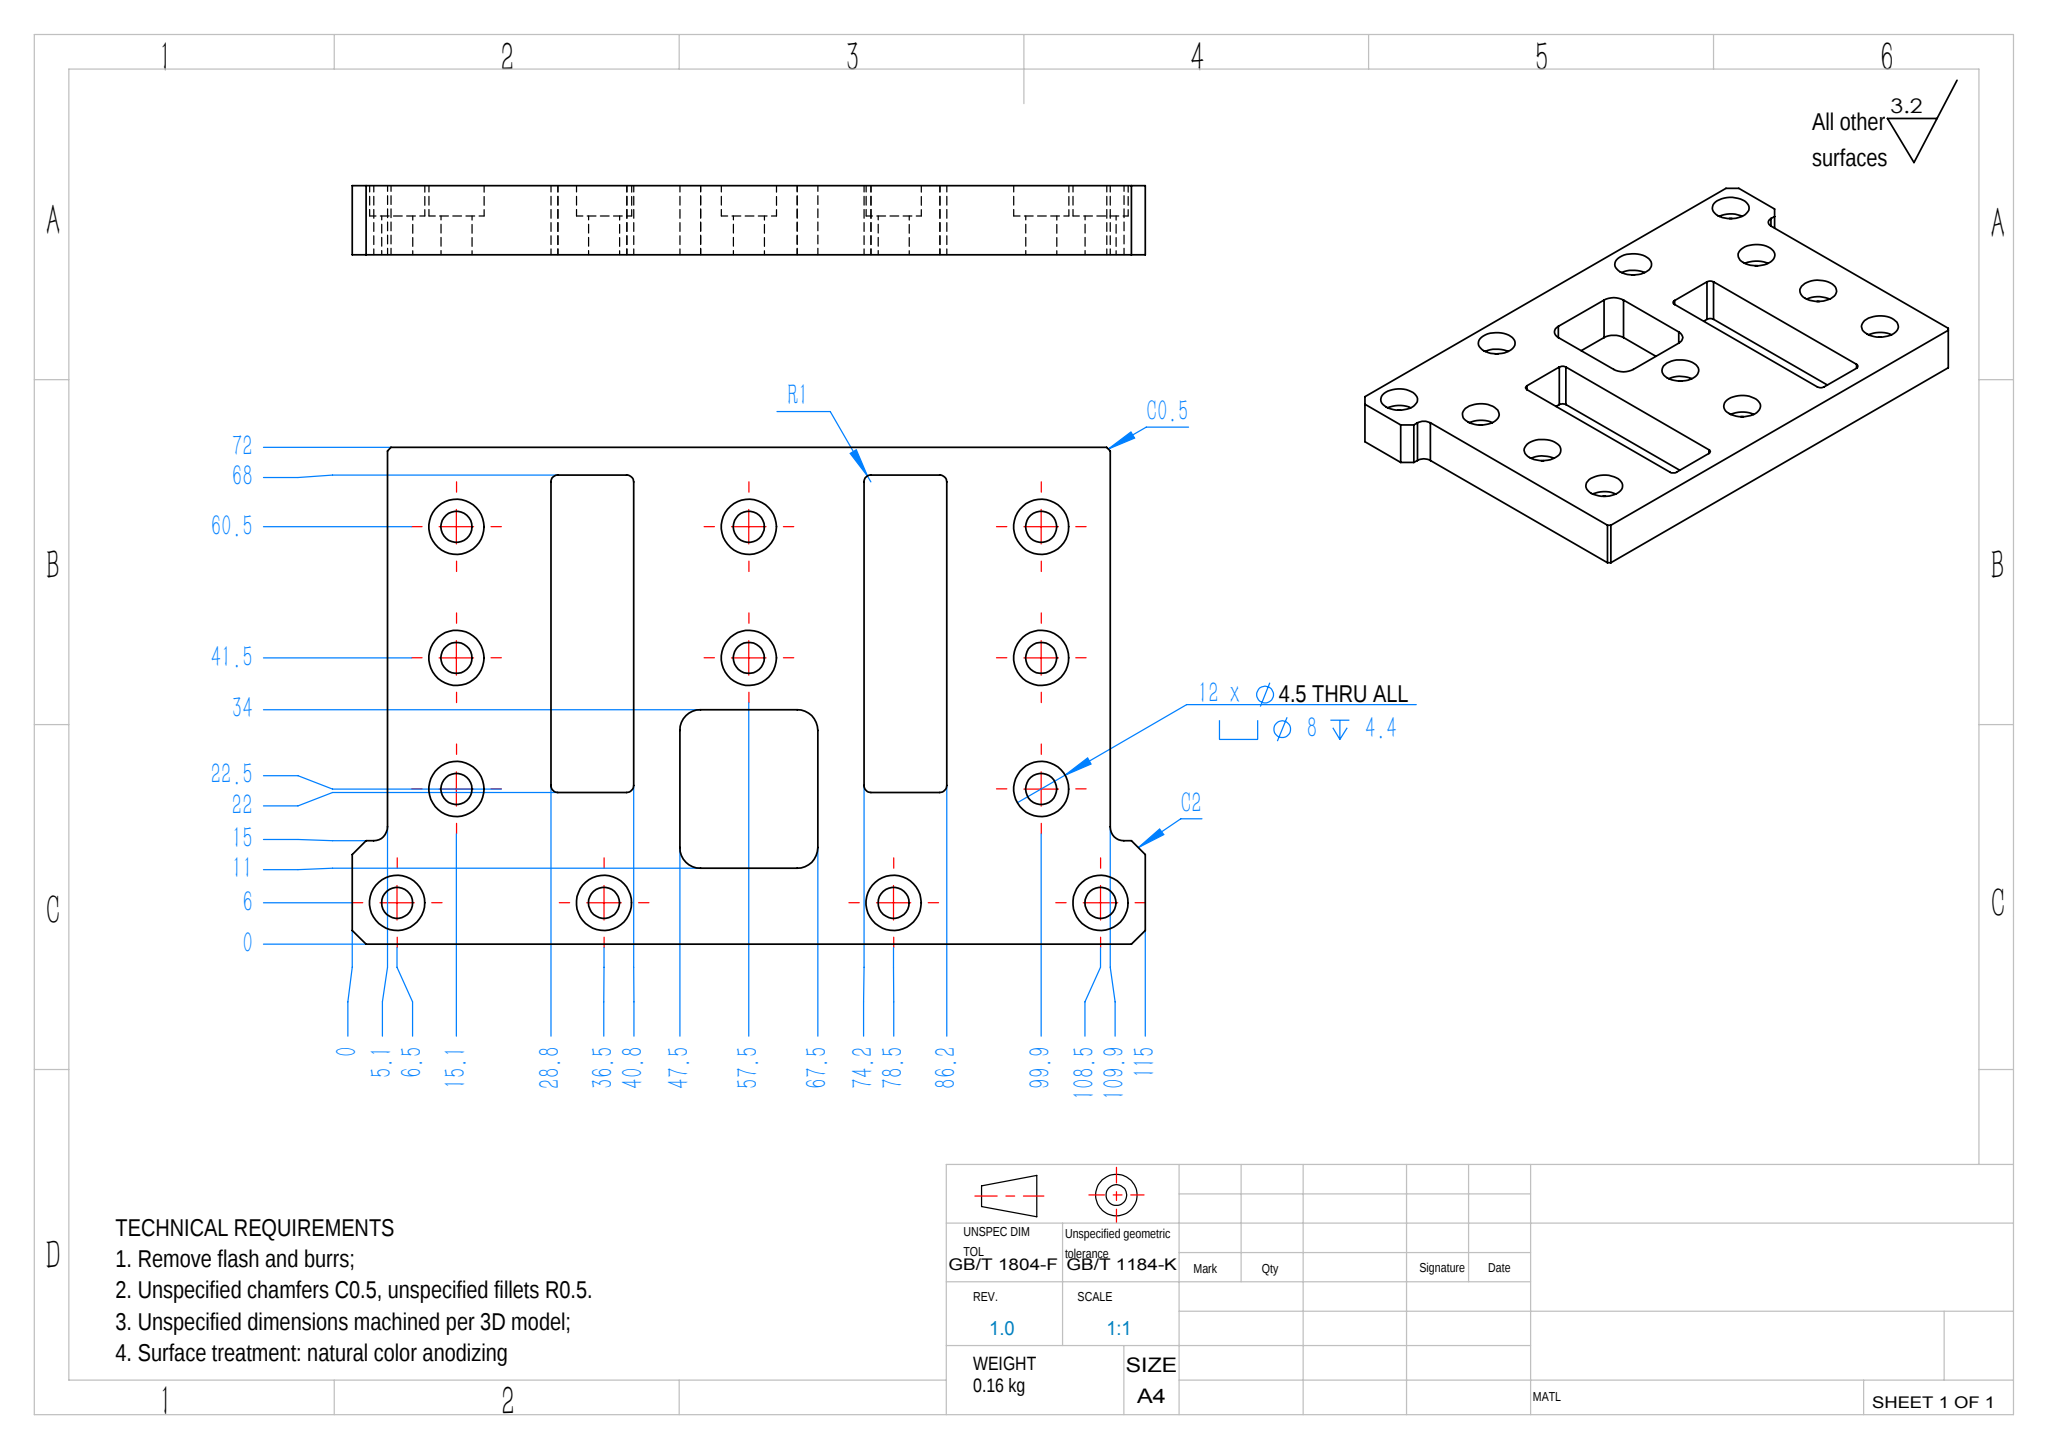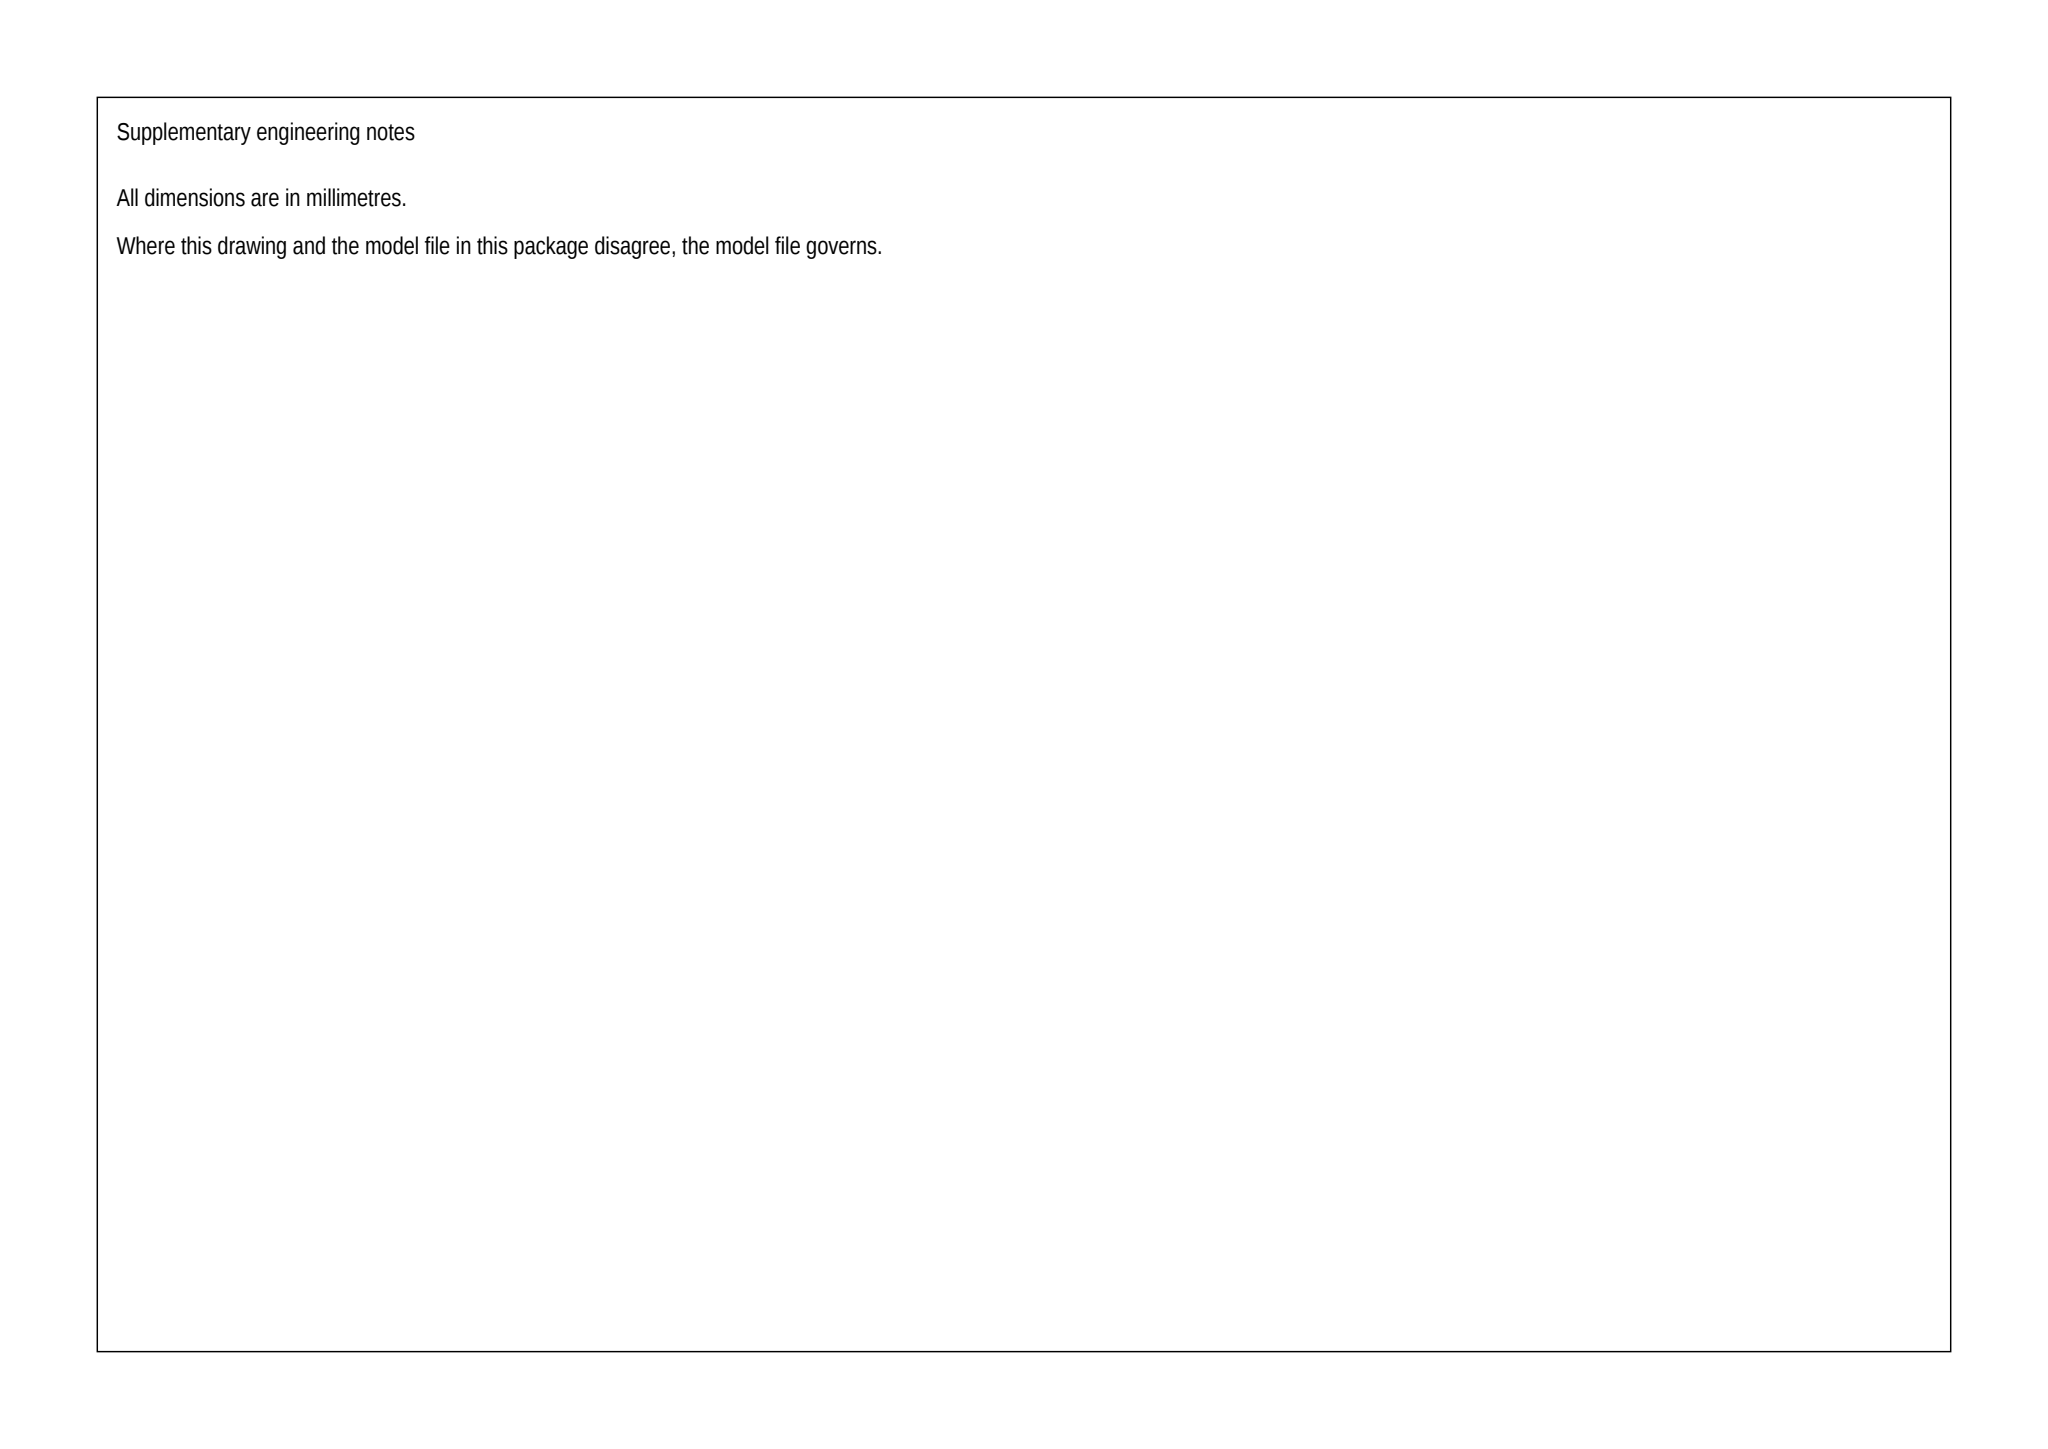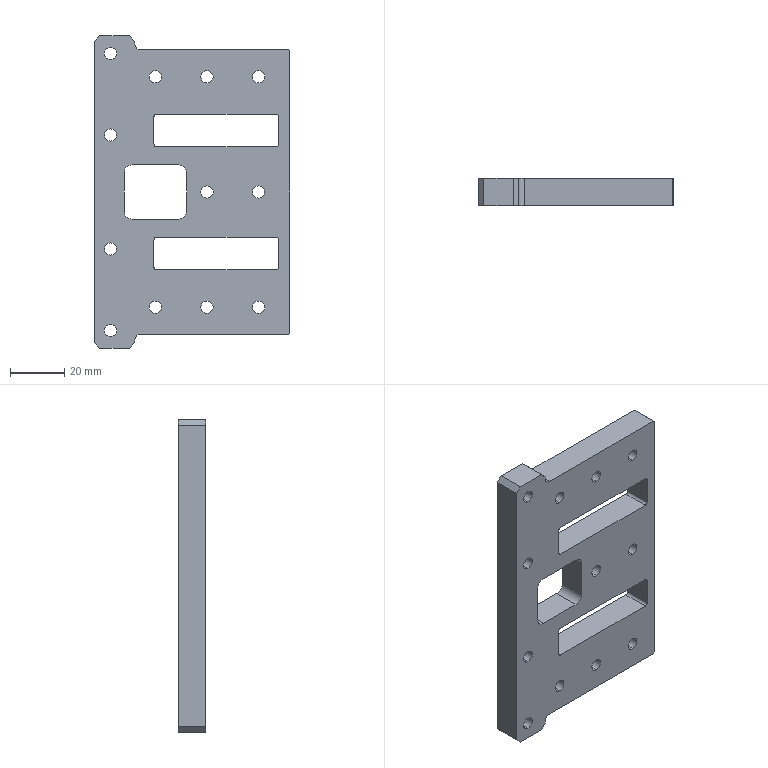Part | SolidWorks | mm | 1 solid | 102 faces | box 72 x 10 x 115 mm | volume 57652 mm3 | cylinder 62 | plane 40 | commonest cylinder face diameters 8 x24 4.5 x24 2 x8 6 x4 4 x2
Drawing notes:
PLATE 115 X 72 X 10 THK | from the solid: bbox_xyz [72,10,115]; y planes only at 0.0 and 10.0
2X EDGE STEP 5.1 DP X 57 HIGH (X15 TO X72), FULL THK | from the solid: z planes 0/5.1 and 109.9/115 (5.1); x planes 15.0 (2) to 72.0 = 57; no mid y plane, full 10 thk
2X R2 AT STEP RE-ENTRANT CNRS (X15 / Z5.1 & Z109.9) | from the solid: Ø4.0 y-axis cyls at (x17,z3.1) and (x17,z111.9), L=10, tangent to x=15 and z=5.1/109.9
C2 AT STEP CNR (X15/Z0 & X15/Z115), 2X | from the solid: C2 called out on sheet 1 at X15/Z115; mirrored x=15 (2) / z=0 & 115 step geometry at both ends
2X SLOT 12 WIDE X 46 LG, R1 ENDS, THRU 10 | from the solid: z planes 28.8/40.8 and 74.2/86.2 = 12 wide; x planes 22/68 = 46 lg; R1 end cyls Ø2 L=10
RND RECT POCKET 23 X 20, R3 CNRS, THRU 10 | from the solid: x planes 11/34 = 23; z planes 47.5/67.5 = 20; Ø6 cnr cyls at x14/31, z50.5/64.5, L=10
build123d program:
from build123d import *

# Parameters (mm, degrees)
SKETCH2_W                                       = 72
SKETCH2_H                                       = 115
BOSS_EXTRUDE1_DEPTH                             = 5
CUT_EXTRUDE3_DEPTH                              = 20
CHAMFER1_SIZE                                   = 2
SKETCH11_W                                      = 57
SKETCH11_H                                      = 5.1
CUT_EXTRUDE4_DEPTH                              = 69.573
M4_HEX_SOCKET_HEAD_CAP_SCREW_CBORE1_D           = 4.5
M4_HEX_SOCKET_HEAD_CAP_SCREW_CBORE1_CBORE_D     = 8
M4_HEX_SOCKET_HEAD_CAP_SCREW_CBORE1_CBORE_DEPTH = 4.4
CHAMFER2_SIZE                                   = 2
CHAMFER3_SIZE                                   = 0.5
FILLET1_R                                       = 2
SKETCH12_W                                      = 23
SKETCH12_H                                      = 20
CUT_EXTRUDE5_DEPTH                              = 69.573
FILLET2_R                                       = 3


with BuildPart() as part:
    # Sketch2 → Boss-Extrude1 (new, symmetric)
    with BuildSketch(Plane(origin=(0, 0, 0), x_dir=(1, 0, 0), z_dir=(0, 1, 0))):
        Rectangle(SKETCH2_W, SKETCH2_H)
    extrude(amount=BOSS_EXTRUDE1_DEPTH, both=True)

    # Sketch5 → Cut-Extrude3 (cut)
    with BuildSketch(Plane.XZ.offset(5)):
        with BuildLine():
            Line((31, -16.7), (-13, -16.7))
            ThreePointArc((-13, -16.7), (-13.707, -16.993), (-14, -17.7))
            Line((-14, -17.7), (-14, -27.7))
            ThreePointArc((-14, -27.7), (-13.707, -28.407), (-13, -28.7))
            Line((-13, -28.7), (31, -28.7))
            ThreePointArc((31, -28.7), (31.707, -28.407), (32, -27.7))
            Line((32, -27.7), (32, -17.7))
            ThreePointArc((32, -17.7), (31.707, -16.993), (31, -16.7))
        make_face()
        with BuildLine():
            Line((-14, 17.7), (-14, 27.7))
            ThreePointArc((-14, 27.7), (-13.707, 28.407), (-13, 28.7))
            Line((-13, 28.7), (31, 28.7))
            ThreePointArc((31, 28.7), (31.707, 28.407), (32, 27.7))
            Line((32, 27.7), (32, 17.7))
            ThreePointArc((32, 17.7), (31.707, 16.993), (31, 16.7))
            Line((31, 16.7), (-13, 16.7))
            ThreePointArc((-13, 16.7), (-13.707, 16.993), (-14, 17.7))
        make_face()
    extrude(amount=-CUT_EXTRUDE3_DEPTH, mode=Mode.SUBTRACT)

    # Chamfer1
    chamfer1_edges = [part.edges().sort_by_distance(p)[0] for p in [
        (-36, 0, 57.5),
        (-36, 0, -57.5),
    ]]
    chamfer(chamfer1_edges, length=CHAMFER1_SIZE)

    # Sketch11 → Cut-Extrude4 (cut, through all)
    with BuildSketch(Plane.XZ.offset(5)):
        with Locations((7.5, 54.95)):
            Rectangle(SKETCH11_W, SKETCH11_H)
        with Locations((7.5, -54.95)):
            Rectangle(SKETCH11_W, SKETCH11_H)
    extrude(amount=-CUT_EXTRUDE4_DEPTH, mode=Mode.SUBTRACT)

    # M4 Hex Socket Head Cap Screw CBORE1 (through all)
    with Locations(Plane(origin=(0, 5, 0), x_dir=(1, 0, 0), z_dir=(0, 1, 0))):
        with Locations((5.5, 42.4), (24.5, 42.4), (-13.5, 42.4), (-30, 51), (5.5, 0), (24.5, 0), (-30, 21), (5.5, -42.4), (24.5, -42.4), (-13.5, -42.4), (-30, -21), (-30, -51)):
            CounterBoreHole(M4_HEX_SOCKET_HEAD_CAP_SCREW_CBORE1_D / 2, M4_HEX_SOCKET_HEAD_CAP_SCREW_CBORE1_CBORE_D / 2, M4_HEX_SOCKET_HEAD_CAP_SCREW_CBORE1_CBORE_DEPTH)

    # Chamfer2
    chamfer2_edges = [part.edges().sort_by_distance(p)[0] for p in [
        (-21, 0, 57.5),
        (-21, 0, -57.5),
    ]]
    chamfer(chamfer2_edges, length=CHAMFER2_SIZE)

    # Chamfer3
    chamfer3_edges = [part.edges().sort_by_distance(p)[0] for p in [
        (36, 0, 52.4),
        (36, 0, -52.4),
    ]]
    chamfer(chamfer3_edges, length=CHAMFER3_SIZE)

    # Fillet1
    fillet1_edges = [part.edges().sort_by_distance(p)[0] for p in [
        (-21, 0, 52.4),
        (-21, 0, -52.4),
    ]]
    fillet(fillet1_edges, radius=FILLET1_R)

    # Sketch12 → Cut-Extrude5 (cut, through all)
    with BuildSketch(Plane(origin=(0, 5, 0), x_dir=(1, 0, 0), z_dir=(0, 1, 0))):
        with Locations((-13.5, 0)):
            Rectangle(SKETCH12_W, SKETCH12_H)
    extrude(amount=-CUT_EXTRUDE5_DEPTH, mode=Mode.SUBTRACT)

    # Fillet2
    fillet2_edges = [part.edges().sort_by_distance(p)[0] for p in [
        (-2, 0, -10),
        (-2, 0, 10),
        (-25, 0, 10),
        (-25, 0, -10),
    ]]
    fillet(fillet2_edges, radius=FILLET2_R)


solid = part.part